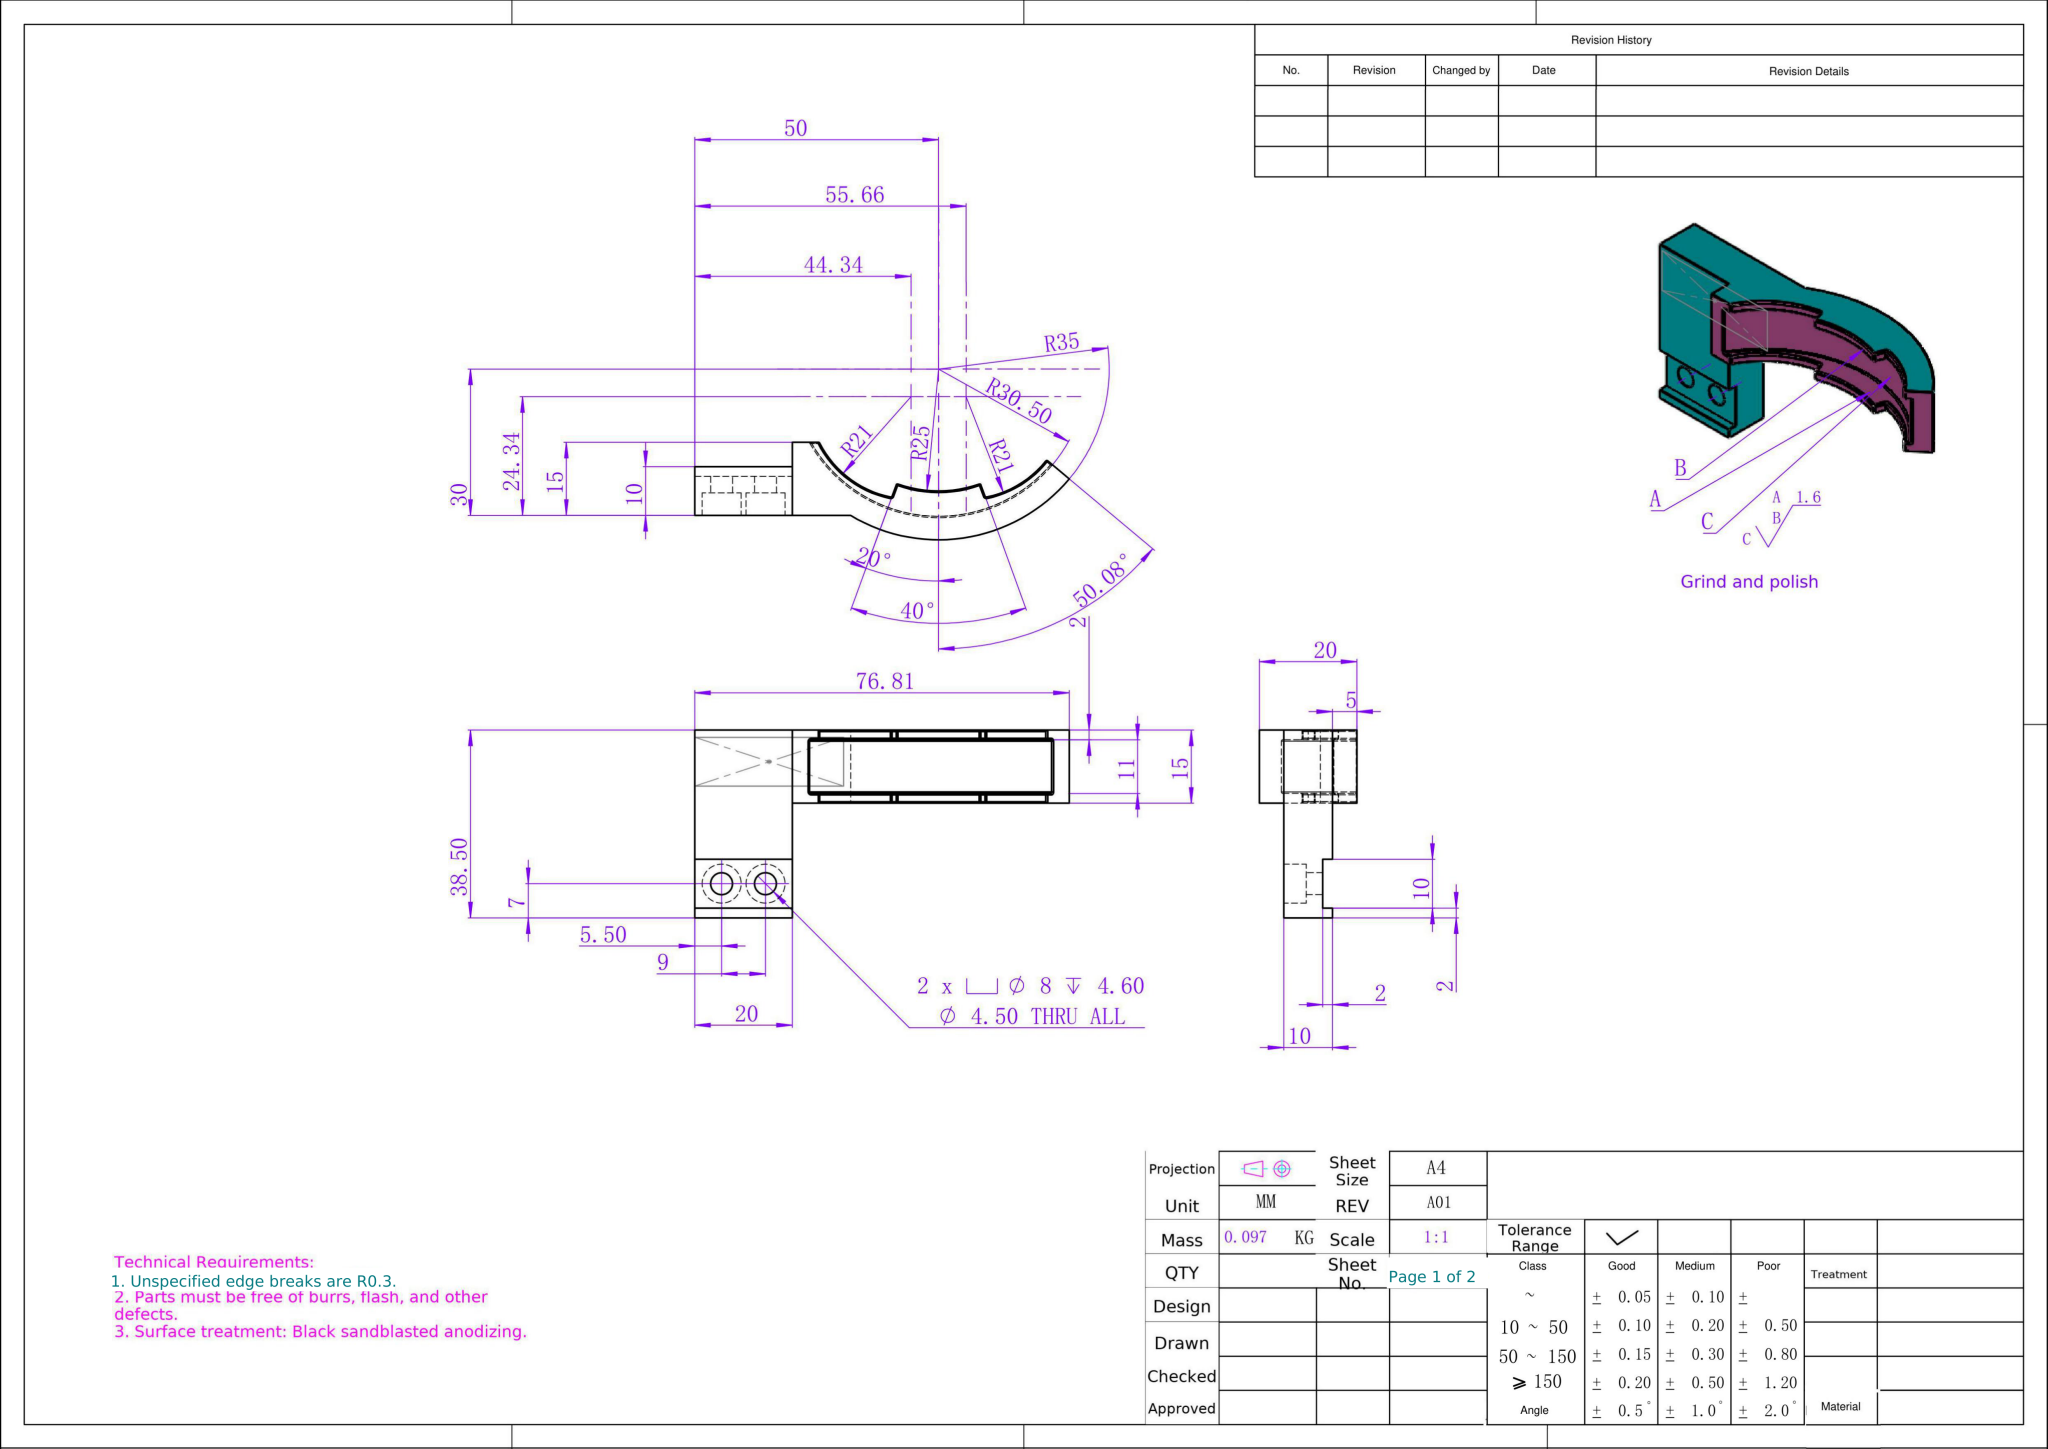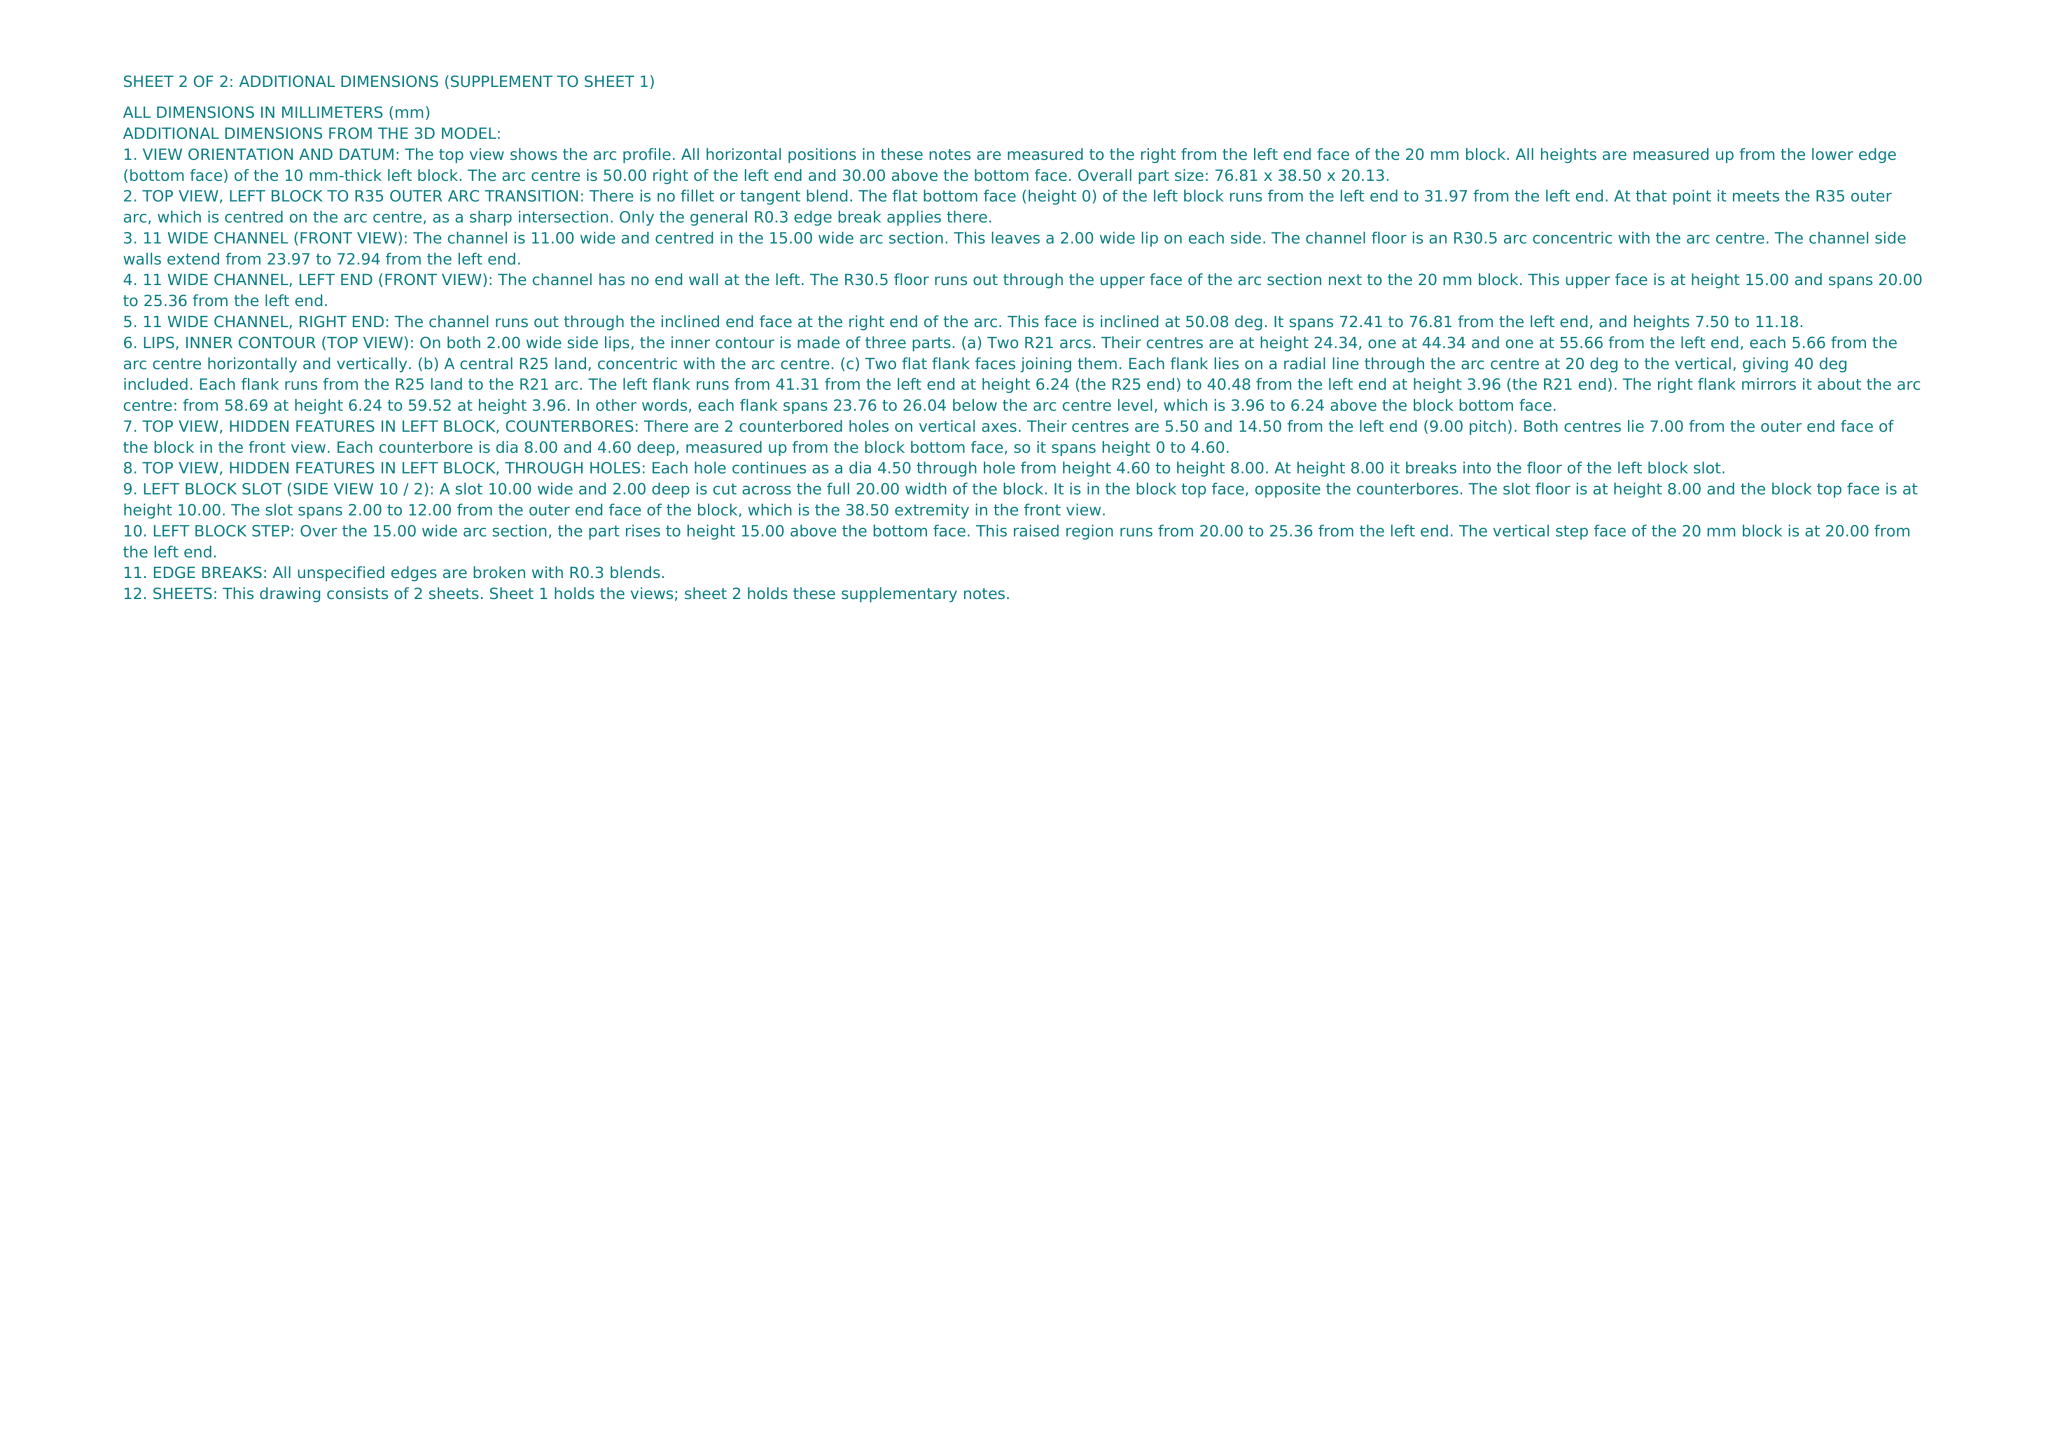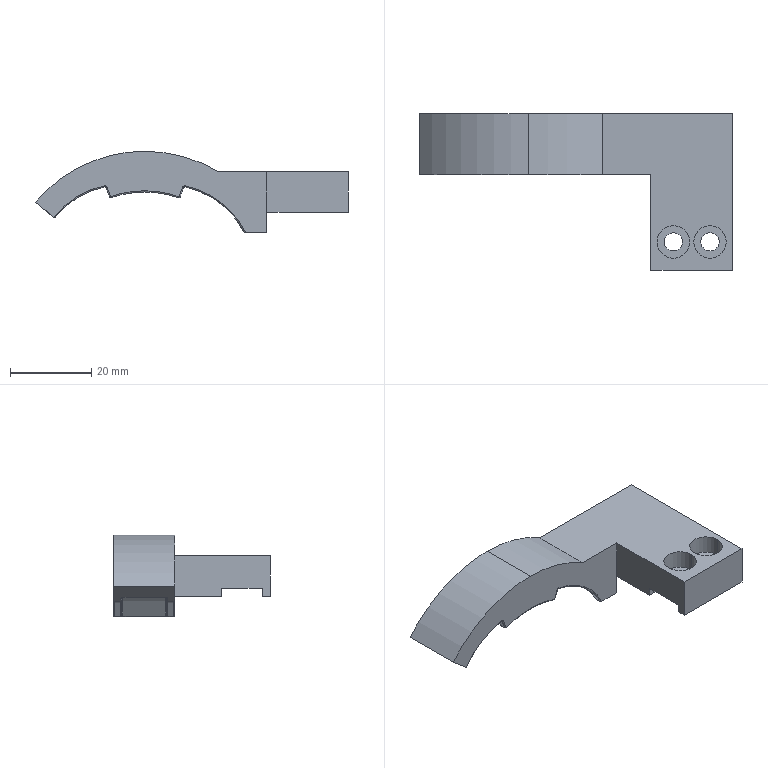Part | NX | mm | 1 solid | 121 faces | box 76.81 x 38.5 x 20 mm | volume 12618 mm3 | cylinder 50 | torus 33 | plane 22 | sphere 12 | spline 4 | commonest cylinder face diameters 0.6 x30 8 x4 4.5 x4 50 x4 42 x4 61 x2 70 x2